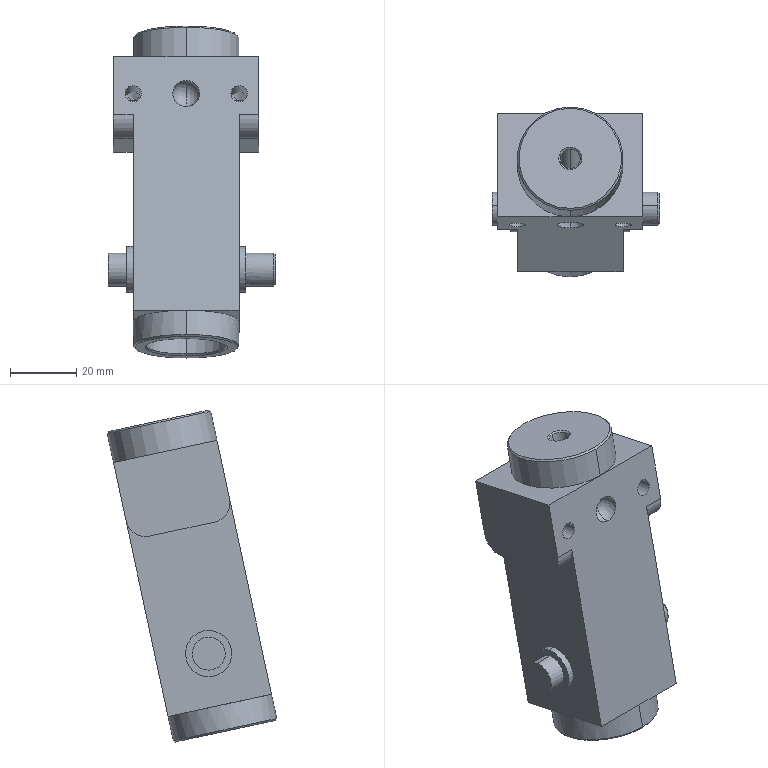Component | SolidWorks | Ornament-2 | 1 solid | 62 faces | volume 75612 mm3 | cylinder 24 | plane 20 | cone 16 | sphere 2 | commonest cylinder face diameters 5 x4 14 x4 10 x4 32 x4 12 x4 6 x2 24 x2